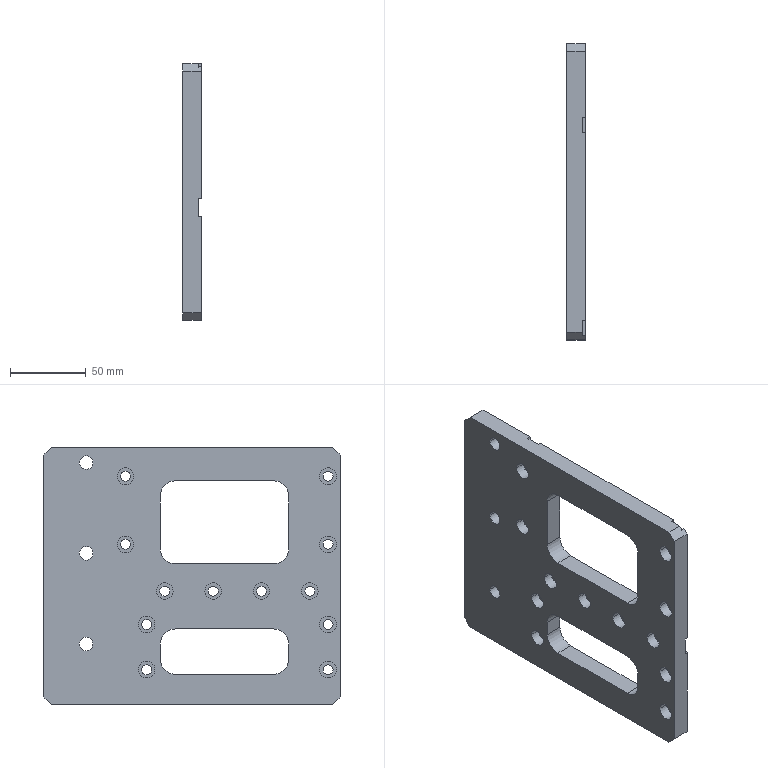Component | SolidWorks | 17081801-804-014A-1 | 1 solid | 104 faces | box 12 x 196 x 170 mm | volume 295000 mm3 | cylinder 62 | plane 42 | commonest cylinder face diameters 11 x24 6.6 x24 20 x8 9 x6 | material AL6061
build123d program:
from build123d import *

# Parameters (mm, degrees)
SKETCH1_W                                       = 136
SKETCH1_H                                       = 170
BOSS_EXTRUDE1_DEPTH                             = 6
M6_HEX_SOCKET_HEAD_CAP_SCREW_CBORE1_D           = 6.6
M6_HEX_SOCKET_HEAD_CAP_SCREW_CBORE1_DEPTH       = 13
M6_HEX_SOCKET_HEAD_CAP_SCREW_CBORE1_CBORE_D     = 11
M6_HEX_SOCKET_HEAD_CAP_SCREW_CBORE1_CBORE_DEPTH = 6.4
M6_HEX_SOCKET_HEAD_CAP_SCREW_CBORE1_TIP         = 1.983
M6_HEX_SOCKET_HEAD_CAP_SCREW_CBORE2_D           = 6.6
M6_HEX_SOCKET_HEAD_CAP_SCREW_CBORE2_DEPTH       = 13
M6_HEX_SOCKET_HEAD_CAP_SCREW_CBORE2_CBORE_D     = 11
M6_HEX_SOCKET_HEAD_CAP_SCREW_CBORE2_CBORE_DEPTH = 6.4
M6_HEX_SOCKET_HEAD_CAP_SCREW_CBORE2_TIP         = 1.983
SKETCH10_W                                      = 12
SKETCH10_H                                      = 170
BOSS_EXTRUDE2_DEPTH                             = 60
LPATTERN1_COUNT                                 = 2
LPATTERN1_PITCH                                 = 45
SKETCH11_W                                      = 85
SKETCH11_H                                      = 55
SKETCH11_H_2                                    = 30
CUT_EXTRUDE1_DEPTH                              = 155.12
FILLET1_R                                       = 10
M8_CLEARANCE_HOLE1_D                            = 9
CHAMFER1_SIZE                                   = 5
M6_HEX_SOCKET_HEAD_CAP_SCREW_CBORE4_D           = 6.6
M6_HEX_SOCKET_HEAD_CAP_SCREW_CBORE4_DEPTH       = 13
M6_HEX_SOCKET_HEAD_CAP_SCREW_CBORE4_CBORE_D     = 11
M6_HEX_SOCKET_HEAD_CAP_SCREW_CBORE4_CBORE_DEPTH = 6.4
M6_HEX_SOCKET_HEAD_CAP_SCREW_CBORE4_TIP         = 1.983
SKETCH14_W                                      = 196
SKETCH14_H                                      = 12
CUT_EXTRUDE2_DEPTH                              = 2
SKETCH16_W                                      = 10
SKETCH16_H                                      = 89
CUT_EXTRUDE4_DEPTH                              = 2


with BuildPart() as part:
    # Sketch1 → Boss-Extrude1 (new, symmetric)
    with BuildSketch(Plane.XY):
        Rectangle(SKETCH1_W, SKETCH1_H)
    extrude(amount=BOSS_EXTRUDE1_DEPTH, both=True)

    # M6 Hex Socket Head Cap Screw CBORE1
    with Locations(Plane.XY.offset(6)):
        with Locations((-48, -10), (-16, -10), (16, -10), (48, -10)):
            CounterBoreHole(M6_HEX_SOCKET_HEAD_CAP_SCREW_CBORE1_D / 2, M6_HEX_SOCKET_HEAD_CAP_SCREW_CBORE1_CBORE_D / 2, M6_HEX_SOCKET_HEAD_CAP_SCREW_CBORE1_CBORE_DEPTH, depth=M6_HEX_SOCKET_HEAD_CAP_SCREW_CBORE1_DEPTH)
            with Locations((0, 0, -(M6_HEX_SOCKET_HEAD_CAP_SCREW_CBORE1_DEPTH + M6_HEX_SOCKET_HEAD_CAP_SCREW_CBORE1_TIP / 2))):  # 118° drill point
                Cone(0, M6_HEX_SOCKET_HEAD_CAP_SCREW_CBORE1_D / 2, M6_HEX_SOCKET_HEAD_CAP_SCREW_CBORE1_TIP, mode=Mode.SUBTRACT)

    # M6 Hex Socket Head Cap Screw CBORE2
    with Locations(Plane.XY.offset(6)):
        with Locations((-60, -32), (-60, -62), (60, -32), (60, -62)):
            CounterBoreHole(M6_HEX_SOCKET_HEAD_CAP_SCREW_CBORE2_D / 2, M6_HEX_SOCKET_HEAD_CAP_SCREW_CBORE2_CBORE_D / 2, M6_HEX_SOCKET_HEAD_CAP_SCREW_CBORE2_CBORE_DEPTH, depth=M6_HEX_SOCKET_HEAD_CAP_SCREW_CBORE2_DEPTH)
            with Locations((0, 0, -(M6_HEX_SOCKET_HEAD_CAP_SCREW_CBORE2_DEPTH + M6_HEX_SOCKET_HEAD_CAP_SCREW_CBORE2_TIP / 2))):  # 118° drill point
                Cone(0, M6_HEX_SOCKET_HEAD_CAP_SCREW_CBORE2_D / 2, M6_HEX_SOCKET_HEAD_CAP_SCREW_CBORE2_TIP, mode=Mode.SUBTRACT)

    # Sketch10 → Boss-Extrude2 (add)
    with BuildSketch(Plane.ZY.offset(68)):
        Rectangle(SKETCH10_W, SKETCH10_H)
    extrude(amount=BOSS_EXTRUDE2_DEPTH)

    # Sketch8 → M6 Hex Socket Head Cap Screw CBORE3 (revolve, cut)
    with BuildSketch(Plane(origin=(-74, 21, 6), x_dir=(0, -1, 0), z_dir=(1, 0, 0))):
        Polygon((0, 0), (0, 14.983), (3.3, 13), (3.3, 6.4), (5.5, 6.4), (5.5, 0), align=None)
    m6_hex_socket_head_cap_screw_cbore3 = revolve(axis=Axis((-74, 21, 12.35), (0, 0, -1)), mode=Mode.SUBTRACT)

    # LPattern1: M6 Hex Socket Head Cap Screw CBORE3 ×2
    with Locations(*[(0, i * LPATTERN1_PITCH, 0) for i in range(1, LPATTERN1_COUNT)]):
        add(m6_hex_socket_head_cap_screw_cbore3, mode=Mode.SUBTRACT)

    # Sketch11 → Cut-Extrude1 (cut, through all)
    with BuildSketch(Plane.XY.offset(6)):
        with Locations((-8.5, 35.5)):
            Rectangle(SKETCH11_W, SKETCH11_H)
        with Locations((-8.5, -50)):
            Rectangle(SKETCH11_W, SKETCH11_H_2)
    extrude(amount=-CUT_EXTRUDE1_DEPTH, mode=Mode.SUBTRACT)

    # Fillet1
    fillet1_edges = [part.edges().sort_by_distance(p)[0] for p in [
        (-51, 8, 0),
        (-51, 63, 0),
        (34, 63, 0),
        (34, 8, 0),
        (-51, -65, 0),
        (-51, -35, 0),
        (34, -35, 0),
        (34, -65, 0),
    ]]
    fillet(fillet1_edges, radius=FILLET1_R)

    # M8 Clearance Hole1 (through all)
    with Locations(Plane.XY.offset(6)):
        with Locations((-100, -45), (-100, 15), (-100, 75)):
            Hole(M8_CLEARANCE_HOLE1_D / 2)

    # Chamfer1
    chamfer1_edges = [part.edges().sort_by_distance(p)[0] for p in [
        (68, 85, 0),
        (68, -85, 0),
        (-128, 85, 0),
        (-128, -85, 0),
    ]]
    chamfer(chamfer1_edges, length=CHAMFER1_SIZE)

    # M6 Hex Socket Head Cap Screw CBORE4
    with Locations(Plane(origin=(62, 0, 6), x_dir=(-1, 0, 0), z_dir=(0, 0, 1))):
        with Locations((2, -21), (2, -66)):
            CounterBoreHole(M6_HEX_SOCKET_HEAD_CAP_SCREW_CBORE4_D / 2, M6_HEX_SOCKET_HEAD_CAP_SCREW_CBORE4_CBORE_D / 2, M6_HEX_SOCKET_HEAD_CAP_SCREW_CBORE4_CBORE_DEPTH, depth=M6_HEX_SOCKET_HEAD_CAP_SCREW_CBORE4_DEPTH)
            with Locations((0, 0, -(M6_HEX_SOCKET_HEAD_CAP_SCREW_CBORE4_DEPTH + M6_HEX_SOCKET_HEAD_CAP_SCREW_CBORE4_TIP / 2))):  # 118° drill point
                Cone(0, M6_HEX_SOCKET_HEAD_CAP_SCREW_CBORE4_D / 2, M6_HEX_SOCKET_HEAD_CAP_SCREW_CBORE4_TIP, mode=Mode.SUBTRACT)

    # Sketch14 → Cut-Extrude2 (cut)
    with BuildSketch(Plane(origin=(0, 0, -6), x_dir=(-1, 0, 0), z_dir=(0, 0, -1))):
        with Locations((30, -10)):
            Rectangle(SKETCH14_W, SKETCH14_H)
    extrude(amount=-CUT_EXTRUDE2_DEPTH, mode=Mode.SUBTRACT)

    # Sketch16 → Cut-Extrude4 (cut)
    with BuildSketch(Plane(origin=(0, 0, -6), x_dir=(-1, 0, 0), z_dir=(0, 0, -1))):
        with Locations((74, 40.5)):
            Rectangle(SKETCH16_W, SKETCH16_H)
        with Locations((-60, 40.5)):
            Rectangle(SKETCH16_W, SKETCH16_H)
    extrude(amount=-CUT_EXTRUDE4_DEPTH, mode=Mode.SUBTRACT)


solid = part.part

# Placed as in the assembly
solid = solid.moved(Location((-120.5, 2034.4, 236), (90, -90, 0)))